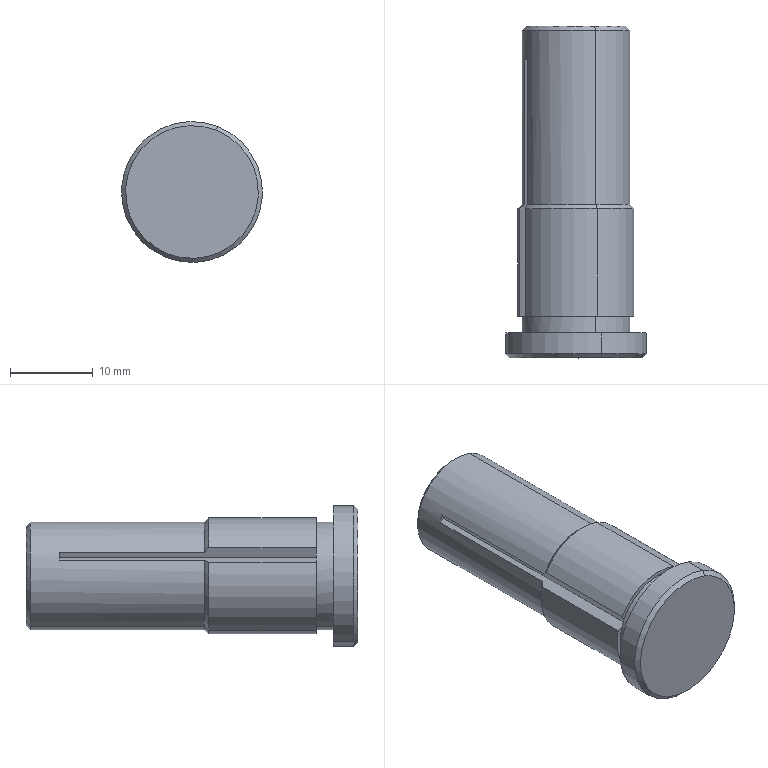Component | SolidWorks | 20-1 | 1 solid | 24 faces | box 17 x 40 x 17 mm | volume 5844 mm3 | cylinder 9 | plane 8 | cone 7 | commonest cylinder face diameters 13 x4 14 x3 17 x2
STEP:
#1=COLOUR_RGB('',0.7922,0.8196,0.9333);
#2=FILL_AREA_STYLE_COLOUR('',#1);
#3=FILL_AREA_STYLE('',(#2));
#4=SURFACE_STYLE_FILL_AREA(#3);
#5=SURFACE_SIDE_STYLE('',(#4));
#6=SURFACE_STYLE_USAGE(.BOTH.,#5);
#7=PRESENTATION_STYLE_ASSIGNMENT((#6));
#8=CARTESIAN_POINT('',(-5.962,10.472,25.382));
#9=VERTEX_POINT('',#8);
#10=CARTESIAN_POINT('',(-6.112,10.472,25.696));
#11=VERTEX_POINT('',#10);
#12=CARTESIAN_POINT('',(-5.868,10.472,25.62));
#13=DIRECTION('',(-0.,1.,-0.));
#14=DIRECTION('',(-0.3666,0.,-0.9304));
#15=AXIS2_PLACEMENT_3D('',#12,#13,#14);
#16=CIRCLE('',#15,0.2559);
#17=EDGE_CURVE('',#9,#11,#16,.T.);
#18=ORIENTED_EDGE('',*,*,#17,.F.);
#19=CARTESIAN_POINT('',(-5.969,10.452,25.364));
#20=VERTEX_POINT('',#19);
#21=CARTESIAN_POINT('',(-5.962,10.472,25.382));
#22=DIRECTION('',(-0.2592,-0.7071,-0.6579));
#23=VECTOR('',#22,39.37);
#24=LINE('',#21,#23);
#25=EDGE_CURVE('',#9,#20,#24,.T.);
#26=ORIENTED_EDGE('',*,*,#25,.T.);
#27=CARTESIAN_POINT('',(-6.135,10.452,25.686));
#28=VERTEX_POINT('',#27);
#29=CARTESIAN_POINT('',(-5.868,10.452,25.62));
#30=DIRECTION('',(0.,-1.,0.));
#31=DIRECTION('',(0.3666,0.,0.9304));
#32=AXIS2_PLACEMENT_3D('',#29,#30,#31);
#33=CIRCLE('',#32,0.2756);
#34=EDGE_CURVE('',#28,#20,#33,.T.);
#35=ORIENTED_EDGE('',*,*,#34,.F.);
#36=CARTESIAN_POINT('',(-6.112,10.472,25.696));
#37=CARTESIAN_POINT('',(-6.12,10.466,25.693));
#38=CARTESIAN_POINT('',(-6.128,10.459,25.689));
#39=CARTESIAN_POINT('',(-6.135,10.452,25.686));
#40=B_SPLINE_CURVE_WITH_KNOTS('',3,(#36,#37,#38,#39),.UNSPECIFIED.,.F.,.F.,(4,4),(0.,0.0008148),.UNSPECIFIED.);
#41=EDGE_CURVE('',#11,#28,#40,.T.);
#42=ORIENTED_EDGE('',*,*,#41,.F.);
#43=EDGE_LOOP('',(#18,#26,#35,#42));
#44=FACE_OUTER_BOUND('',#43,.T.);
#45=CARTESIAN_POINT('',(-5.868,10.472,25.62));
#46=DIRECTION('',(0.,-1.,0.));
#47=DIRECTION('',(0.3666,0.,0.9304));
#48=AXIS2_PLACEMENT_3D('',#45,#46,#47);
#49=CONICAL_SURFACE('',#48,0.2559,0.7854);
#50=ADVANCED_FACE('',(#44),#49,.T.);
#51=ORIENTED_EDGE('',*,*,#25,.F.);
#52=CARTESIAN_POINT('',(-5.774,10.472,25.858));
#53=VERTEX_POINT('',#52);
#54=CARTESIAN_POINT('',(-5.868,10.472,25.62));
#55=DIRECTION('',(-0.,1.,-0.));
#56=DIRECTION('',(-0.3666,0.,-0.9304));
#57=AXIS2_PLACEMENT_3D('',#54,#55,#56);
#58=CIRCLE('',#57,0.2559);
#59=EDGE_CURVE('',#53,#9,#58,.T.);
#60=ORIENTED_EDGE('',*,*,#59,.F.);
#61=CARTESIAN_POINT('',(-5.767,10.452,25.877));
#62=VERTEX_POINT('',#61);
#63=CARTESIAN_POINT('',(-5.774,10.472,25.858));
#64=DIRECTION('',(0.2592,-0.7071,0.6579));
#65=VECTOR('',#64,39.37);
#66=LINE('',#63,#65);
#67=EDGE_CURVE('',#53,#62,#66,.T.);
#68=ORIENTED_EDGE('',*,*,#67,.T.);
#69=CARTESIAN_POINT('',(-5.868,10.452,25.62));
#70=DIRECTION('',(0.,-1.,0.));
#71=DIRECTION('',(0.3666,0.,0.9304));
#72=AXIS2_PLACEMENT_3D('',#69,#70,#71);
#73=CIRCLE('',#72,0.2756);
#74=EDGE_CURVE('',#20,#62,#73,.T.);
#75=ORIENTED_EDGE('',*,*,#74,.F.);
#76=EDGE_LOOP('',(#51,#60,#68,#75));
#77=FACE_OUTER_BOUND('',#76,.T.);
#78=CARTESIAN_POINT('',(-5.868,10.472,25.62));
#79=DIRECTION('',(0.,-1.,0.));
#80=DIRECTION('',(0.3666,0.,0.9304));
#81=AXIS2_PLACEMENT_3D('',#78,#79,#80);
#82=CONICAL_SURFACE('',#81,0.2559,0.7854);
#83=ADVANCED_FACE('',(#77),#82,.T.);
#84=CARTESIAN_POINT('',(-5.752,9.744,25.913));
#85=VERTEX_POINT('',#84);
#86=CARTESIAN_POINT('',(-5.983,9.744,25.327));
#87=VERTEX_POINT('',#86);
#88=CARTESIAN_POINT('',(-5.868,9.744,25.62));
#89=DIRECTION('',(0.,-1.,0.));
#90=DIRECTION('',(-0.3666,0.,-0.9304));
#91=AXIS2_PLACEMENT_3D('',#88,#89,#90);
#92=CIRCLE('',#91,0.315);
#93=EDGE_CURVE('',#85,#87,#92,.T.);
#94=ORIENTED_EDGE('',*,*,#93,.F.);
#95=CARTESIAN_POINT('',(-5.745,9.763,25.931));
#96=VERTEX_POINT('',#95);
#97=CARTESIAN_POINT('',(-5.745,9.763,25.931));
#98=DIRECTION('',(0.2592,0.7071,0.6579));
#99=VECTOR('',#98,39.37);
#100=LINE('',#97,#99);
#101=EDGE_CURVE('',#85,#96,#100,.T.);
#102=ORIENTED_EDGE('',*,*,#101,.T.);
#103=CARTESIAN_POINT('',(-5.99,9.763,25.309));
#104=VERTEX_POINT('',#103);
#105=CARTESIAN_POINT('',(-5.868,9.763,25.62));
#106=DIRECTION('',(-0.,1.,-0.));
#107=DIRECTION('',(-0.3666,0.,-0.9304));
#108=AXIS2_PLACEMENT_3D('',#105,#106,#107);
#109=CIRCLE('',#108,0.3346);
#110=EDGE_CURVE('',#104,#96,#109,.T.);
#111=ORIENTED_EDGE('',*,*,#110,.F.);
#112=CARTESIAN_POINT('',(-5.99,9.763,25.309));
#113=DIRECTION('',(-0.2592,0.7071,-0.6579));
#114=VECTOR('',#113,39.37);
#115=LINE('',#112,#114);
#116=EDGE_CURVE('',#87,#104,#115,.T.);
#117=ORIENTED_EDGE('',*,*,#116,.F.);
#118=EDGE_LOOP('',(#94,#102,#111,#117));
#119=FACE_OUTER_BOUND('',#118,.T.);
#120=CARTESIAN_POINT('',(-5.868,9.763,25.62));
#121=DIRECTION('',(-0.,1.,-0.));
#122=DIRECTION('',(-0.3666,0.,-0.9304));
#123=AXIS2_PLACEMENT_3D('',#120,#121,#122);
#124=CONICAL_SURFACE('',#123,0.3346,0.7854);
#125=ADVANCED_FACE('',(#119),#124,.T.);
#126=CARTESIAN_POINT('',(-5.954,11.319,25.4));
#127=VERTEX_POINT('',#126);
#128=CARTESIAN_POINT('',(-5.781,11.319,25.84));
#129=VERTEX_POINT('',#128);
#130=CARTESIAN_POINT('',(-5.868,11.319,25.62));
#131=DIRECTION('',(-0.,1.,-0.));
#132=DIRECTION('',(0.3666,0.,0.9304));
#133=AXIS2_PLACEMENT_3D('',#130,#131,#132);
#134=CIRCLE('',#133,0.2362);
#135=EDGE_CURVE('',#127,#129,#134,.T.);
#136=ORIENTED_EDGE('',*,*,#135,.F.);
#137=CARTESIAN_POINT('',(-5.962,11.299,25.382));
#138=VERTEX_POINT('',#137);
#139=CARTESIAN_POINT('',(-5.954,11.319,25.4));
#140=DIRECTION('',(-0.2592,-0.7071,-0.6579));
#141=VECTOR('',#140,39.37);
#142=LINE('',#139,#141);
#143=EDGE_CURVE('',#127,#138,#142,.T.);
#144=ORIENTED_EDGE('',*,*,#143,.T.);
#145=CARTESIAN_POINT('',(-5.774,11.299,25.858));
#146=VERTEX_POINT('',#145);
#147=CARTESIAN_POINT('',(-5.868,11.299,25.62));
#148=DIRECTION('',(0.,-1.,0.));
#149=DIRECTION('',(0.3666,0.,0.9304));
#150=AXIS2_PLACEMENT_3D('',#147,#148,#149);
#151=CIRCLE('',#150,0.2559);
#152=EDGE_CURVE('',#146,#138,#151,.T.);
#153=ORIENTED_EDGE('',*,*,#152,.F.);
#154=CARTESIAN_POINT('',(-5.781,11.319,25.84));
#155=DIRECTION('',(0.2592,-0.7071,0.6579));
#156=VECTOR('',#155,39.37);
#157=LINE('',#154,#156);
#158=EDGE_CURVE('',#129,#146,#157,.T.);
#159=ORIENTED_EDGE('',*,*,#158,.F.);
#160=EDGE_LOOP('',(#136,#144,#153,#159));
#161=FACE_OUTER_BOUND('',#160,.T.);
#162=CARTESIAN_POINT('',(-5.868,11.319,25.62));
#163=DIRECTION('',(0.,-1.,0.));
#164=DIRECTION('',(0.3666,0.,0.9304));
#165=AXIS2_PLACEMENT_3D('',#162,#163,#164);
#166=CONICAL_SURFACE('',#165,0.2362,0.7854);
#167=ADVANCED_FACE('',(#161),#166,.T.);
#168=CARTESIAN_POINT('',(-5.962,9.862,25.382));
#169=VERTEX_POINT('',#168);
#170=CARTESIAN_POINT('',(-5.774,9.862,25.858));
#171=VERTEX_POINT('',#170);
#172=CARTESIAN_POINT('',(-5.868,9.862,25.62));
#173=DIRECTION('',(-0.,1.,-0.));
#174=DIRECTION('',(-0.3666,0.,-0.9304));
#175=AXIS2_PLACEMENT_3D('',#172,#173,#174);
#176=CIRCLE('',#175,0.2559);
#177=EDGE_CURVE('',#169,#171,#176,.T.);
#178=ORIENTED_EDGE('',*,*,#177,.T.);
#179=CARTESIAN_POINT('',(-5.774,9.941,25.858));
#180=VERTEX_POINT('',#179);
#181=CARTESIAN_POINT('',(-5.774,11.319,25.858));
#182=DIRECTION('',(-0.,1.,-0.));
#183=VECTOR('',#182,39.37);
#184=LINE('',#181,#183);
#185=EDGE_CURVE('',#171,#180,#184,.T.);
#186=ORIENTED_EDGE('',*,*,#185,.T.);
#187=CARTESIAN_POINT('',(-6.098,9.941,25.731));
#188=VERTEX_POINT('',#187);
#189=CARTESIAN_POINT('',(-5.868,9.941,25.62));
#190=DIRECTION('',(-0.,1.,-0.));
#191=DIRECTION('',(-0.3666,0.,-0.9304));
#192=AXIS2_PLACEMENT_3D('',#189,#190,#191);
#193=CIRCLE('',#192,0.2559);
#194=EDGE_CURVE('',#188,#180,#193,.T.);
#195=ORIENTED_EDGE('',*,*,#194,.F.);
#196=CARTESIAN_POINT('',(-6.112,9.941,25.696));
#197=VERTEX_POINT('',#196);
#198=CARTESIAN_POINT('',(-5.868,9.941,25.62));
#199=DIRECTION('',(-0.,1.,-0.));
#200=DIRECTION('',(-0.3666,0.,-0.9304));
#201=AXIS2_PLACEMENT_3D('',#198,#199,#200);
#202=CIRCLE('',#201,0.2559);
#203=EDGE_CURVE('',#197,#188,#202,.T.);
#204=ORIENTED_EDGE('',*,*,#203,.F.);
#205=CARTESIAN_POINT('',(-5.962,9.941,25.382));
#206=VERTEX_POINT('',#205);
#207=CARTESIAN_POINT('',(-5.868,9.941,25.62));
#208=DIRECTION('',(-0.,1.,-0.));
#209=DIRECTION('',(-0.3666,0.,-0.9304));
#210=AXIS2_PLACEMENT_3D('',#207,#208,#209);
#211=CIRCLE('',#210,0.2559);
#212=EDGE_CURVE('',#206,#197,#211,.T.);
#213=ORIENTED_EDGE('',*,*,#212,.F.);
#214=CARTESIAN_POINT('',(-5.962,11.319,25.382));
#215=DIRECTION('',(-0.,1.,-0.));
#216=VECTOR('',#215,39.37);
#217=LINE('',#214,#216);
#218=EDGE_CURVE('',#169,#206,#217,.T.);
#219=ORIENTED_EDGE('',*,*,#218,.F.);
#220=EDGE_LOOP('',(#178,#186,#195,#204,#213,#219));
#221=FACE_OUTER_BOUND('',#220,.T.);
#222=CARTESIAN_POINT('',(-5.868,11.319,25.62));
#223=DIRECTION('',(-0.,1.,-0.));
#224=DIRECTION('',(-0.3666,0.,-0.9304));
#225=AXIS2_PLACEMENT_3D('',#222,#223,#224);
#226=CYLINDRICAL_SURFACE('',#225,0.2559);
#227=ADVANCED_FACE('',(#221),#226,.T.);
#228=ORIENTED_EDGE('',*,*,#110,.T.);
#229=CARTESIAN_POINT('',(-5.745,9.862,25.931));
#230=VERTEX_POINT('',#229);
#231=CARTESIAN_POINT('',(-5.745,11.319,25.931));
#232=DIRECTION('',(-0.,1.,-0.));
#233=VECTOR('',#232,39.37);
#234=LINE('',#231,#233);
#235=EDGE_CURVE('',#96,#230,#234,.T.);
#236=ORIENTED_EDGE('',*,*,#235,.T.);
#237=CARTESIAN_POINT('',(-5.99,9.862,25.309));
#238=VERTEX_POINT('',#237);
#239=CARTESIAN_POINT('',(-5.868,9.862,25.62));
#240=DIRECTION('',(-0.,1.,-0.));
#241=DIRECTION('',(-0.3666,0.,-0.9304));
#242=AXIS2_PLACEMENT_3D('',#239,#240,#241);
#243=CIRCLE('',#242,0.3346);
#244=EDGE_CURVE('',#238,#230,#243,.T.);
#245=ORIENTED_EDGE('',*,*,#244,.F.);
#246=CARTESIAN_POINT('',(-5.99,11.319,25.309));
#247=DIRECTION('',(-0.,1.,-0.));
#248=VECTOR('',#247,39.37);
#249=LINE('',#246,#248);
#250=EDGE_CURVE('',#104,#238,#249,.T.);
#251=ORIENTED_EDGE('',*,*,#250,.F.);
#252=EDGE_LOOP('',(#228,#236,#245,#251));
#253=FACE_OUTER_BOUND('',#252,.T.);
#254=CARTESIAN_POINT('',(-5.868,11.319,25.62));
#255=DIRECTION('',(-0.,1.,-0.));
#256=DIRECTION('',(-0.3666,0.,-0.9304));
#257=AXIS2_PLACEMENT_3D('',#254,#255,#256);
#258=CYLINDRICAL_SURFACE('',#257,0.3346);
#259=ADVANCED_FACE('',(#253),#258,.T.);
#260=CARTESIAN_POINT('',(-6.098,10.472,25.731));
#261=VERTEX_POINT('',#260);
#262=CARTESIAN_POINT('',(-5.868,10.472,25.62));
#263=DIRECTION('',(-0.,1.,-0.));
#264=DIRECTION('',(-0.3666,0.,-0.9304));
#265=AXIS2_PLACEMENT_3D('',#262,#263,#264);
#266=CIRCLE('',#265,0.2559);
#267=EDGE_CURVE('',#261,#53,#266,.T.);
#268=ORIENTED_EDGE('',*,*,#267,.T.);
#269=CARTESIAN_POINT('',(-5.774,11.319,25.858));
#270=DIRECTION('',(-0.,1.,-0.));
#271=VECTOR('',#270,39.37);
#272=LINE('',#269,#271);
#273=EDGE_CURVE('',#53,#146,#272,.T.);
#274=ORIENTED_EDGE('',*,*,#273,.T.);
#275=ORIENTED_EDGE('',*,*,#152,.T.);
#276=CARTESIAN_POINT('',(-5.962,11.319,25.382));
#277=DIRECTION('',(-0.,1.,-0.));
#278=VECTOR('',#277,39.37);
#279=LINE('',#276,#278);
#280=EDGE_CURVE('',#9,#138,#279,.T.);
#281=ORIENTED_EDGE('',*,*,#280,.F.);
#282=ORIENTED_EDGE('',*,*,#17,.T.);
#283=CARTESIAN_POINT('',(-6.112,11.161,25.696));
#284=VERTEX_POINT('',#283);
#285=CARTESIAN_POINT('',(-6.112,11.319,25.696));
#286=DIRECTION('',(0.,-1.,0.));
#287=VECTOR('',#286,39.37);
#288=LINE('',#285,#287);
#289=EDGE_CURVE('',#284,#11,#288,.T.);
#290=ORIENTED_EDGE('',*,*,#289,.F.);
#291=CARTESIAN_POINT('',(-6.098,11.161,25.731));
#292=VERTEX_POINT('',#291);
#293=CARTESIAN_POINT('',(-5.868,11.161,25.62));
#294=DIRECTION('',(0.,-1.,0.));
#295=DIRECTION('',(0.9304,0.,-0.3666));
#296=AXIS2_PLACEMENT_3D('',#293,#294,#295);
#297=CIRCLE('',#296,0.2559);
#298=EDGE_CURVE('',#292,#284,#297,.T.);
#299=ORIENTED_EDGE('',*,*,#298,.F.);
#300=CARTESIAN_POINT('',(-6.098,11.319,25.731));
#301=DIRECTION('',(0.,-1.,0.));
#302=VECTOR('',#301,39.37);
#303=LINE('',#300,#302);
#304=EDGE_CURVE('',#292,#261,#303,.T.);
#305=ORIENTED_EDGE('',*,*,#304,.T.);
#306=EDGE_LOOP('',(#268,#274,#275,#281,#282,#290,#299,#305));
#307=FACE_OUTER_BOUND('',#306,.T.);
#308=CARTESIAN_POINT('',(-5.868,11.319,25.62));
#309=DIRECTION('',(-0.,1.,-0.));
#310=DIRECTION('',(-0.3666,0.,-0.9304));
#311=AXIS2_PLACEMENT_3D('',#308,#309,#310);
#312=CYLINDRICAL_SURFACE('',#311,0.2559);
#313=ADVANCED_FACE('',(#307),#312,.T.);
#314=CARTESIAN_POINT('',(-6.108,9.941,25.755));
#315=VERTEX_POINT('',#314);
#316=CARTESIAN_POINT('',(-5.767,9.941,25.877));
#317=VERTEX_POINT('',#316);
#318=CARTESIAN_POINT('',(-5.868,9.941,25.62));
#319=DIRECTION('',(-0.,1.,-0.));
#320=DIRECTION('',(-0.3666,0.,-0.9304));
#321=AXIS2_PLACEMENT_3D('',#318,#319,#320);
#322=CIRCLE('',#321,0.2756);
#323=EDGE_CURVE('',#315,#317,#322,.T.);
#324=ORIENTED_EDGE('',*,*,#323,.T.);
#325=CARTESIAN_POINT('',(-5.767,11.319,25.877));
#326=DIRECTION('',(-0.,1.,-0.));
#327=VECTOR('',#326,39.37);
#328=LINE('',#325,#327);
#329=EDGE_CURVE('',#317,#62,#328,.T.);
#330=ORIENTED_EDGE('',*,*,#329,.T.);
#331=CARTESIAN_POINT('',(-6.108,10.452,25.755));
#332=VERTEX_POINT('',#331);
#333=CARTESIAN_POINT('',(-5.868,10.452,25.62));
#334=DIRECTION('',(0.,-1.,0.));
#335=DIRECTION('',(0.3666,0.,0.9304));
#336=AXIS2_PLACEMENT_3D('',#333,#334,#335);
#337=CIRCLE('',#336,0.2756);
#338=EDGE_CURVE('',#62,#332,#337,.T.);
#339=ORIENTED_EDGE('',*,*,#338,.T.);
#340=CARTESIAN_POINT('',(-6.108,11.319,25.755));
#341=DIRECTION('',(0.,-1.,0.));
#342=VECTOR('',#341,39.37);
#343=LINE('',#340,#342);
#344=EDGE_CURVE('',#332,#315,#343,.T.);
#345=ORIENTED_EDGE('',*,*,#344,.T.);
#346=EDGE_LOOP('',(#324,#330,#339,#345));
#347=FACE_OUTER_BOUND('',#346,.T.);
#348=CARTESIAN_POINT('',(-5.868,11.319,25.62));
#349=DIRECTION('',(-0.,1.,-0.));
#350=DIRECTION('',(-0.3666,0.,-0.9304));
#351=AXIS2_PLACEMENT_3D('',#348,#349,#350);
#352=CYLINDRICAL_SURFACE('',#351,0.2756);
#353=ADVANCED_FACE('',(#347),#352,.T.);
#354=ORIENTED_EDGE('',*,*,#329,.F.);
#355=CARTESIAN_POINT('',(-5.969,9.941,25.364));
#356=VERTEX_POINT('',#355);
#357=CARTESIAN_POINT('',(-5.868,9.941,25.62));
#358=DIRECTION('',(-0.,1.,-0.));
#359=DIRECTION('',(-0.3666,0.,-0.9304));
#360=AXIS2_PLACEMENT_3D('',#357,#358,#359);
#361=CIRCLE('',#360,0.2756);
#362=EDGE_CURVE('',#317,#356,#361,.T.);
#363=ORIENTED_EDGE('',*,*,#362,.T.);
#364=CARTESIAN_POINT('',(-5.969,11.319,25.364));
#365=DIRECTION('',(-0.,1.,-0.));
#366=VECTOR('',#365,39.37);
#367=LINE('',#364,#366);
#368=EDGE_CURVE('',#356,#20,#367,.T.);
#369=ORIENTED_EDGE('',*,*,#368,.T.);
#370=ORIENTED_EDGE('',*,*,#74,.T.);
#371=EDGE_LOOP('',(#354,#363,#369,#370));
#372=FACE_OUTER_BOUND('',#371,.T.);
#373=CARTESIAN_POINT('',(-5.868,11.319,25.62));
#374=DIRECTION('',(-0.,1.,-0.));
#375=DIRECTION('',(-0.3666,0.,-0.9304));
#376=AXIS2_PLACEMENT_3D('',#373,#374,#375);
#377=CYLINDRICAL_SURFACE('',#376,0.2756);
#378=ADVANCED_FACE('',(#372),#377,.T.);
#379=CARTESIAN_POINT('',(-6.135,9.941,25.686));
#380=VERTEX_POINT('',#379);
#381=CARTESIAN_POINT('',(-5.934,9.941,25.773));
#382=DIRECTION('',(-0.9171,-0.,-0.3987));
#383=VECTOR('',#382,39.37);
#384=LINE('',#381,#383);
#385=EDGE_CURVE('',#197,#380,#384,.T.);
#386=ORIENTED_EDGE('',*,*,#385,.T.);
#387=CARTESIAN_POINT('',(-5.868,9.941,25.62));
#388=DIRECTION('',(-0.,1.,-0.));
#389=DIRECTION('',(-0.3666,0.,-0.9304));
#390=AXIS2_PLACEMENT_3D('',#387,#388,#389);
#391=CIRCLE('',#390,0.2756);
#392=EDGE_CURVE('',#356,#380,#391,.T.);
#393=ORIENTED_EDGE('',*,*,#392,.F.);
#394=ORIENTED_EDGE('',*,*,#362,.F.);
#395=ORIENTED_EDGE('',*,*,#323,.F.);
#396=CARTESIAN_POINT('',(-6.021,9.941,25.554));
#397=DIRECTION('',(-0.3987,0.,0.9171));
#398=VECTOR('',#397,39.37);
#399=LINE('',#396,#398);
#400=EDGE_CURVE('',#188,#315,#399,.T.);
#401=ORIENTED_EDGE('',*,*,#400,.F.);
#402=ORIENTED_EDGE('',*,*,#194,.T.);
#403=CARTESIAN_POINT('',(-5.868,9.941,25.62));
#404=DIRECTION('',(-0.,1.,-0.));
#405=DIRECTION('',(-0.3666,0.,-0.9304));
#406=AXIS2_PLACEMENT_3D('',#403,#404,#405);
#407=CIRCLE('',#406,0.2559);
#408=EDGE_CURVE('',#180,#206,#407,.T.);
#409=ORIENTED_EDGE('',*,*,#408,.T.);
#410=ORIENTED_EDGE('',*,*,#212,.T.);
#411=EDGE_LOOP('',(#386,#393,#394,#395,#401,#402,#409,#410));
#412=FACE_OUTER_BOUND('',#411,.T.);
#413=CARTESIAN_POINT('',(-5.774,9.941,25.858));
#414=DIRECTION('',(-0.,1.,-0.));
#415=DIRECTION('',(-0.3666,-0.,-0.9304));
#416=AXIS2_PLACEMENT_3D('',#413,#414,#415);
#417=PLANE('',#416);
#418=ADVANCED_FACE('',(#412),#417,.F.);
#419=ORIENTED_EDGE('',*,*,#368,.F.);
#420=ORIENTED_EDGE('',*,*,#392,.T.);
#421=CARTESIAN_POINT('',(-6.135,11.319,25.686));
#422=DIRECTION('',(0.,-1.,0.));
#423=VECTOR('',#422,39.37);
#424=LINE('',#421,#423);
#425=EDGE_CURVE('',#28,#380,#424,.T.);
#426=ORIENTED_EDGE('',*,*,#425,.F.);
#427=ORIENTED_EDGE('',*,*,#34,.T.);
#428=EDGE_LOOP('',(#419,#420,#426,#427));
#429=FACE_OUTER_BOUND('',#428,.T.);
#430=CARTESIAN_POINT('',(-5.868,11.319,25.62));
#431=DIRECTION('',(-0.,1.,-0.));
#432=DIRECTION('',(-0.3666,0.,-0.9304));
#433=AXIS2_PLACEMENT_3D('',#430,#431,#432);
#434=CYLINDRICAL_SURFACE('',#433,0.2756);
#435=ADVANCED_FACE('',(#429),#434,.T.);
#436=ORIENTED_EDGE('',*,*,#273,.F.);
#437=ORIENTED_EDGE('',*,*,#59,.T.);
#438=ORIENTED_EDGE('',*,*,#280,.T.);
#439=CARTESIAN_POINT('',(-5.868,11.299,25.62));
#440=DIRECTION('',(0.,-1.,0.));
#441=DIRECTION('',(0.3666,0.,0.9304));
#442=AXIS2_PLACEMENT_3D('',#439,#440,#441);
#443=CIRCLE('',#442,0.2559);
#444=EDGE_CURVE('',#138,#146,#443,.T.);
#445=ORIENTED_EDGE('',*,*,#444,.T.);
#446=EDGE_LOOP('',(#436,#437,#438,#445));
#447=FACE_OUTER_BOUND('',#446,.T.);
#448=CARTESIAN_POINT('',(-5.868,11.319,25.62));
#449=DIRECTION('',(-0.,1.,-0.));
#450=DIRECTION('',(-0.3666,0.,-0.9304));
#451=AXIS2_PLACEMENT_3D('',#448,#449,#450);
#452=CYLINDRICAL_SURFACE('',#451,0.2559);
#453=ADVANCED_FACE('',(#447),#452,.T.);
#454=CARTESIAN_POINT('',(-5.868,9.744,25.62));
#455=DIRECTION('',(0.,-1.,0.));
#456=DIRECTION('',(-0.3666,0.,-0.9304));
#457=AXIS2_PLACEMENT_3D('',#454,#455,#456);
#458=CIRCLE('',#457,0.315);
#459=EDGE_CURVE('',#87,#85,#458,.T.);
#460=ORIENTED_EDGE('',*,*,#459,.T.);
#461=ORIENTED_EDGE('',*,*,#93,.T.);
#462=EDGE_LOOP('',(#460,#461));
#463=FACE_OUTER_BOUND('',#462,.T.);
#464=CARTESIAN_POINT('',(-5.868,9.744,25.62));
#465=DIRECTION('',(-0.,1.,-0.));
#466=DIRECTION('',(-0.3666,-0.,-0.9304));
#467=AXIS2_PLACEMENT_3D('',#464,#465,#466);
#468=PLANE('',#467);
#469=ADVANCED_FACE('',(#463),#468,.F.);
#470=ORIENTED_EDGE('',*,*,#235,.F.);
#471=CARTESIAN_POINT('',(-5.868,9.763,25.62));
#472=DIRECTION('',(-0.,1.,-0.));
#473=DIRECTION('',(-0.3666,0.,-0.9304));
#474=AXIS2_PLACEMENT_3D('',#471,#472,#473);
#475=CIRCLE('',#474,0.3346);
#476=EDGE_CURVE('',#96,#104,#475,.T.);
#477=ORIENTED_EDGE('',*,*,#476,.T.);
#478=ORIENTED_EDGE('',*,*,#250,.T.);
#479=CARTESIAN_POINT('',(-5.868,9.862,25.62));
#480=DIRECTION('',(-0.,1.,-0.));
#481=DIRECTION('',(-0.3666,0.,-0.9304));
#482=AXIS2_PLACEMENT_3D('',#479,#480,#481);
#483=CIRCLE('',#482,0.3346);
#484=EDGE_CURVE('',#230,#238,#483,.T.);
#485=ORIENTED_EDGE('',*,*,#484,.F.);
#486=EDGE_LOOP('',(#470,#477,#478,#485));
#487=FACE_OUTER_BOUND('',#486,.T.);
#488=CARTESIAN_POINT('',(-5.868,11.319,25.62));
#489=DIRECTION('',(-0.,1.,-0.));
#490=DIRECTION('',(-0.3666,0.,-0.9304));
#491=AXIS2_PLACEMENT_3D('',#488,#489,#490);
#492=CYLINDRICAL_SURFACE('',#491,0.3346);
#493=ADVANCED_FACE('',(#487),#492,.T.);
#494=ORIENTED_EDGE('',*,*,#177,.F.);
#495=CARTESIAN_POINT('',(-5.868,9.862,25.62));
#496=DIRECTION('',(-0.,1.,-0.));
#497=DIRECTION('',(-0.3666,0.,-0.9304));
#498=AXIS2_PLACEMENT_3D('',#495,#496,#497);
#499=CIRCLE('',#498,0.2559);
#500=EDGE_CURVE('',#171,#169,#499,.T.);
#501=ORIENTED_EDGE('',*,*,#500,.F.);
#502=EDGE_LOOP('',(#494,#501));
#503=FACE_BOUND('',#502,.T.);
#504=ORIENTED_EDGE('',*,*,#244,.T.);
#505=ORIENTED_EDGE('',*,*,#484,.T.);
#506=EDGE_LOOP('',(#504,#505));
#507=FACE_OUTER_BOUND('',#506,.T.);
#508=CARTESIAN_POINT('',(-5.745,9.862,25.931));
#509=DIRECTION('',(0.,-1.,0.));
#510=DIRECTION('',(0.3666,0.,0.9304));
#511=AXIS2_PLACEMENT_3D('',#508,#509,#510);
#512=PLANE('',#511);
#513=ADVANCED_FACE('',(#503,#507),#512,.F.);
#514=ORIENTED_EDGE('',*,*,#185,.F.);
#515=ORIENTED_EDGE('',*,*,#500,.T.);
#516=ORIENTED_EDGE('',*,*,#218,.T.);
#517=ORIENTED_EDGE('',*,*,#408,.F.);
#518=EDGE_LOOP('',(#514,#515,#516,#517));
#519=FACE_OUTER_BOUND('',#518,.T.);
#520=CARTESIAN_POINT('',(-5.868,11.319,25.62));
#521=DIRECTION('',(-0.,1.,-0.));
#522=DIRECTION('',(-0.3666,0.,-0.9304));
#523=AXIS2_PLACEMENT_3D('',#520,#521,#522);
#524=CYLINDRICAL_SURFACE('',#523,0.2559);
#525=ADVANCED_FACE('',(#519),#524,.T.);
#526=CARTESIAN_POINT('',(-5.868,11.319,25.62));
#527=DIRECTION('',(-0.,1.,-0.));
#528=DIRECTION('',(0.3666,0.,0.9304));
#529=AXIS2_PLACEMENT_3D('',#526,#527,#528);
#530=CIRCLE('',#529,0.2362);
#531=EDGE_CURVE('',#129,#127,#530,.T.);
#532=ORIENTED_EDGE('',*,*,#531,.T.);
#533=ORIENTED_EDGE('',*,*,#135,.T.);
#534=EDGE_LOOP('',(#532,#533));
#535=FACE_OUTER_BOUND('',#534,.T.);
#536=CARTESIAN_POINT('',(-5.774,11.319,25.858));
#537=DIRECTION('',(0.,-1.,0.));
#538=DIRECTION('',(0.3666,0.,0.9304));
#539=AXIS2_PLACEMENT_3D('',#536,#537,#538);
#540=PLANE('',#539);
#541=ADVANCED_FACE('',(#535),#540,.F.);
#542=CARTESIAN_POINT('',(-6.088,9.941,25.707));
#543=VERTEX_POINT('',#542);
#544=CARTESIAN_POINT('',(-6.021,9.941,25.554));
#545=DIRECTION('',(-0.3987,0.,0.9171));
#546=VECTOR('',#545,39.37);
#547=LINE('',#544,#546);
#548=EDGE_CURVE('',#543,#188,#547,.T.);
#549=ORIENTED_EDGE('',*,*,#548,.F.);
#550=CARTESIAN_POINT('',(-5.934,9.941,25.773));
#551=DIRECTION('',(-0.9171,-0.,-0.3987));
#552=VECTOR('',#551,39.37);
#553=LINE('',#550,#552);
#554=EDGE_CURVE('',#543,#197,#553,.T.);
#555=ORIENTED_EDGE('',*,*,#554,.T.);
#556=ORIENTED_EDGE('',*,*,#203,.T.);
#557=EDGE_LOOP('',(#549,#555,#556));
#558=FACE_OUTER_BOUND('',#557,.T.);
#559=CARTESIAN_POINT('',(-5.868,9.941,25.62));
#560=DIRECTION('',(0.,-1.,0.));
#561=DIRECTION('',(0.9304,0.,-0.3666));
#562=AXIS2_PLACEMENT_3D('',#559,#560,#561);
#563=PLANE('',#562);
#564=ADVANCED_FACE('',(#558),#563,.F.);
#565=ORIENTED_EDGE('',*,*,#289,.T.);
#566=ORIENTED_EDGE('',*,*,#41,.T.);
#567=ORIENTED_EDGE('',*,*,#425,.T.);
#568=ORIENTED_EDGE('',*,*,#385,.F.);
#569=ORIENTED_EDGE('',*,*,#554,.F.);
#570=CARTESIAN_POINT('',(-6.088,11.161,25.707));
#571=VERTEX_POINT('',#570);
#572=CARTESIAN_POINT('',(-6.088,11.161,25.707));
#573=DIRECTION('',(0.,-1.,0.));
#574=VECTOR('',#573,39.37);
#575=LINE('',#572,#574);
#576=EDGE_CURVE('',#571,#543,#575,.T.);
#577=ORIENTED_EDGE('',*,*,#576,.F.);
#578=CARTESIAN_POINT('',(-5.934,11.161,25.773));
#579=DIRECTION('',(-0.9171,-0.,-0.3987));
#580=VECTOR('',#579,39.37);
#581=LINE('',#578,#580);
#582=EDGE_CURVE('',#571,#284,#581,.T.);
#583=ORIENTED_EDGE('',*,*,#582,.T.);
#584=EDGE_LOOP('',(#565,#566,#567,#568,#569,#577,#583));
#585=FACE_OUTER_BOUND('',#584,.T.);
#586=CARTESIAN_POINT('',(-5.934,11.161,25.773));
#587=DIRECTION('',(-0.3987,0.,0.9171));
#588=DIRECTION('',(-0.9171,-0.,-0.3987));
#589=AXIS2_PLACEMENT_3D('',#586,#587,#588);
#590=PLANE('',#589);
#591=ADVANCED_FACE('',(#585),#590,.T.);
#592=ORIENTED_EDGE('',*,*,#344,.F.);
#593=CARTESIAN_POINT('',(-6.108,10.452,25.755));
#594=CARTESIAN_POINT('',(-6.105,10.459,25.747));
#595=CARTESIAN_POINT('',(-6.102,10.466,25.739));
#596=CARTESIAN_POINT('',(-6.098,10.472,25.731));
#597=B_SPLINE_CURVE_WITH_KNOTS('',3,(#593,#594,#595,#596),.UNSPECIFIED.,.F.,.F.,(4,4),(0.,0.0008148),.UNSPECIFIED.);
#598=EDGE_CURVE('',#332,#261,#597,.T.);
#599=ORIENTED_EDGE('',*,*,#598,.T.);
#600=ORIENTED_EDGE('',*,*,#304,.F.);
#601=CARTESIAN_POINT('',(-6.021,11.161,25.554));
#602=DIRECTION('',(-0.3987,0.,0.9171));
#603=VECTOR('',#602,39.37);
#604=LINE('',#601,#603);
#605=EDGE_CURVE('',#571,#292,#604,.T.);
#606=ORIENTED_EDGE('',*,*,#605,.F.);
#607=ORIENTED_EDGE('',*,*,#576,.T.);
#608=ORIENTED_EDGE('',*,*,#548,.T.);
#609=ORIENTED_EDGE('',*,*,#400,.T.);
#610=EDGE_LOOP('',(#592,#599,#600,#606,#607,#608,#609));
#611=FACE_OUTER_BOUND('',#610,.T.);
#612=CARTESIAN_POINT('',(-6.021,11.161,25.554));
#613=DIRECTION('',(0.9171,0.,0.3987));
#614=DIRECTION('',(-0.3987,0.,0.9171));
#615=AXIS2_PLACEMENT_3D('',#612,#613,#614);
#616=PLANE('',#615);
#617=ADVANCED_FACE('',(#611),#616,.F.);
#618=ORIENTED_EDGE('',*,*,#298,.T.);
#619=ORIENTED_EDGE('',*,*,#582,.F.);
#620=ORIENTED_EDGE('',*,*,#605,.T.);
#621=EDGE_LOOP('',(#618,#619,#620));
#622=FACE_OUTER_BOUND('',#621,.T.);
#623=CARTESIAN_POINT('',(-5.868,11.161,25.62));
#624=DIRECTION('',(0.,-1.,0.));
#625=DIRECTION('',(0.9304,0.,-0.3666));
#626=AXIS2_PLACEMENT_3D('',#623,#624,#625);
#627=PLANE('',#626);
#628=ADVANCED_FACE('',(#622),#627,.T.);
#629=ORIENTED_EDGE('',*,*,#143,.F.);
#630=ORIENTED_EDGE('',*,*,#531,.F.);
#631=ORIENTED_EDGE('',*,*,#158,.T.);
#632=ORIENTED_EDGE('',*,*,#444,.F.);
#633=EDGE_LOOP('',(#629,#630,#631,#632));
#634=FACE_OUTER_BOUND('',#633,.T.);
#635=CARTESIAN_POINT('',(-5.868,11.319,25.62));
#636=DIRECTION('',(0.,-1.,0.));
#637=DIRECTION('',(0.3666,0.,0.9304));
#638=AXIS2_PLACEMENT_3D('',#635,#636,#637);
#639=CONICAL_SURFACE('',#638,0.2362,0.7854);
#640=ADVANCED_FACE('',(#634),#639,.T.);
#641=ORIENTED_EDGE('',*,*,#101,.F.);
#642=ORIENTED_EDGE('',*,*,#459,.F.);
#643=ORIENTED_EDGE('',*,*,#116,.T.);
#644=ORIENTED_EDGE('',*,*,#476,.F.);
#645=EDGE_LOOP('',(#641,#642,#643,#644));
#646=FACE_OUTER_BOUND('',#645,.T.);
#647=CARTESIAN_POINT('',(-5.868,9.763,25.62));
#648=DIRECTION('',(-0.,1.,-0.));
#649=DIRECTION('',(-0.3666,0.,-0.9304));
#650=AXIS2_PLACEMENT_3D('',#647,#648,#649);
#651=CONICAL_SURFACE('',#650,0.3346,0.7854);
#652=ADVANCED_FACE('',(#646),#651,.T.);
#653=ORIENTED_EDGE('',*,*,#67,.F.);
#654=ORIENTED_EDGE('',*,*,#267,.F.);
#655=ORIENTED_EDGE('',*,*,#598,.F.);
#656=ORIENTED_EDGE('',*,*,#338,.F.);
#657=EDGE_LOOP('',(#653,#654,#655,#656));
#658=FACE_OUTER_BOUND('',#657,.T.);
#659=CARTESIAN_POINT('',(-5.868,10.472,25.62));
#660=DIRECTION('',(0.,-1.,0.));
#661=DIRECTION('',(0.3666,0.,0.9304));
#662=AXIS2_PLACEMENT_3D('',#659,#660,#661);
#663=CONICAL_SURFACE('',#662,0.2559,0.7854);
#664=ADVANCED_FACE('',(#658),#663,.T.);
#665=CLOSED_SHELL('',(#50,#83,#125,#167,#227,#259,#313,#353,#378,#418,#435,#453,#469,#493,#513,#525,#541,#564,#591,#617,#628,#640,#652,#664));
#666=MANIFOLD_SOLID_BREP('',#665);
#667=STYLED_ITEM('',(#7),#666);
#668=(LENGTH_UNIT()NAMED_UNIT(*)SI_UNIT($,.METRE.));
#669=LENGTH_MEASURE_WITH_UNIT(LENGTH_MEASURE(0.0254),#668);
#670=DIMENSIONAL_EXPONENTS(1.,0.,0.,0.,0.,0.,0.);
#671=(CONVERSION_BASED_UNIT('',#669)LENGTH_UNIT()NAMED_UNIT(#670));
#672=UNCERTAINTY_MEASURE_WITH_UNIT(LENGTH_MEASURE(0.00001),#671,'','');
#673=(NAMED_UNIT(*)PLANE_ANGLE_UNIT()SI_UNIT($,.RADIAN.));
#674=(NAMED_UNIT(*)SI_UNIT($,.STERADIAN.)SOLID_ANGLE_UNIT());
#675=(GEOMETRIC_REPRESENTATION_CONTEXT(3)GLOBAL_UNCERTAINTY_ASSIGNED_CONTEXT((#672))GLOBAL_UNIT_ASSIGNED_CONTEXT((#671,#673,#674))REPRESENTATION_CONTEXT('',''));
#676=MECHANICAL_DESIGN_GEOMETRIC_PRESENTATION_REPRESENTATION('',(#667),#675);
#677=CARTESIAN_POINT('',(0.,0.,0.));
#678=DIRECTION('',(0.,0.,1.));
#679=DIRECTION('',(1.,0.,0.));
#680=AXIS2_PLACEMENT_3D('',#677,#678,#679);
#681=(LENGTH_UNIT()NAMED_UNIT(*)SI_UNIT($,.METRE.));
#682=LENGTH_MEASURE_WITH_UNIT(LENGTH_MEASURE(0.0254),#681);
#683=DIMENSIONAL_EXPONENTS(1.,0.,0.,0.,0.,0.,0.);
#684=(CONVERSION_BASED_UNIT('',#682)LENGTH_UNIT()NAMED_UNIT(#683));
#685=UNCERTAINTY_MEASURE_WITH_UNIT(LENGTH_MEASURE(0.00001),#684,'','');
#686=(NAMED_UNIT(*)PLANE_ANGLE_UNIT()SI_UNIT($,.RADIAN.));
#687=(NAMED_UNIT(*)SI_UNIT($,.STERADIAN.)SOLID_ANGLE_UNIT());
#688=(GEOMETRIC_REPRESENTATION_CONTEXT(3)GLOBAL_UNCERTAINTY_ASSIGNED_CONTEXT((#685))GLOBAL_UNIT_ASSIGNED_CONTEXT((#684,#686,#687))REPRESENTATION_CONTEXT('',''));
#689=ADVANCED_BREP_SHAPE_REPRESENTATION('',(#666,#680),#688);
#690=PRESENTATION_LAYER_ASSIGNMENT('','',(#667));